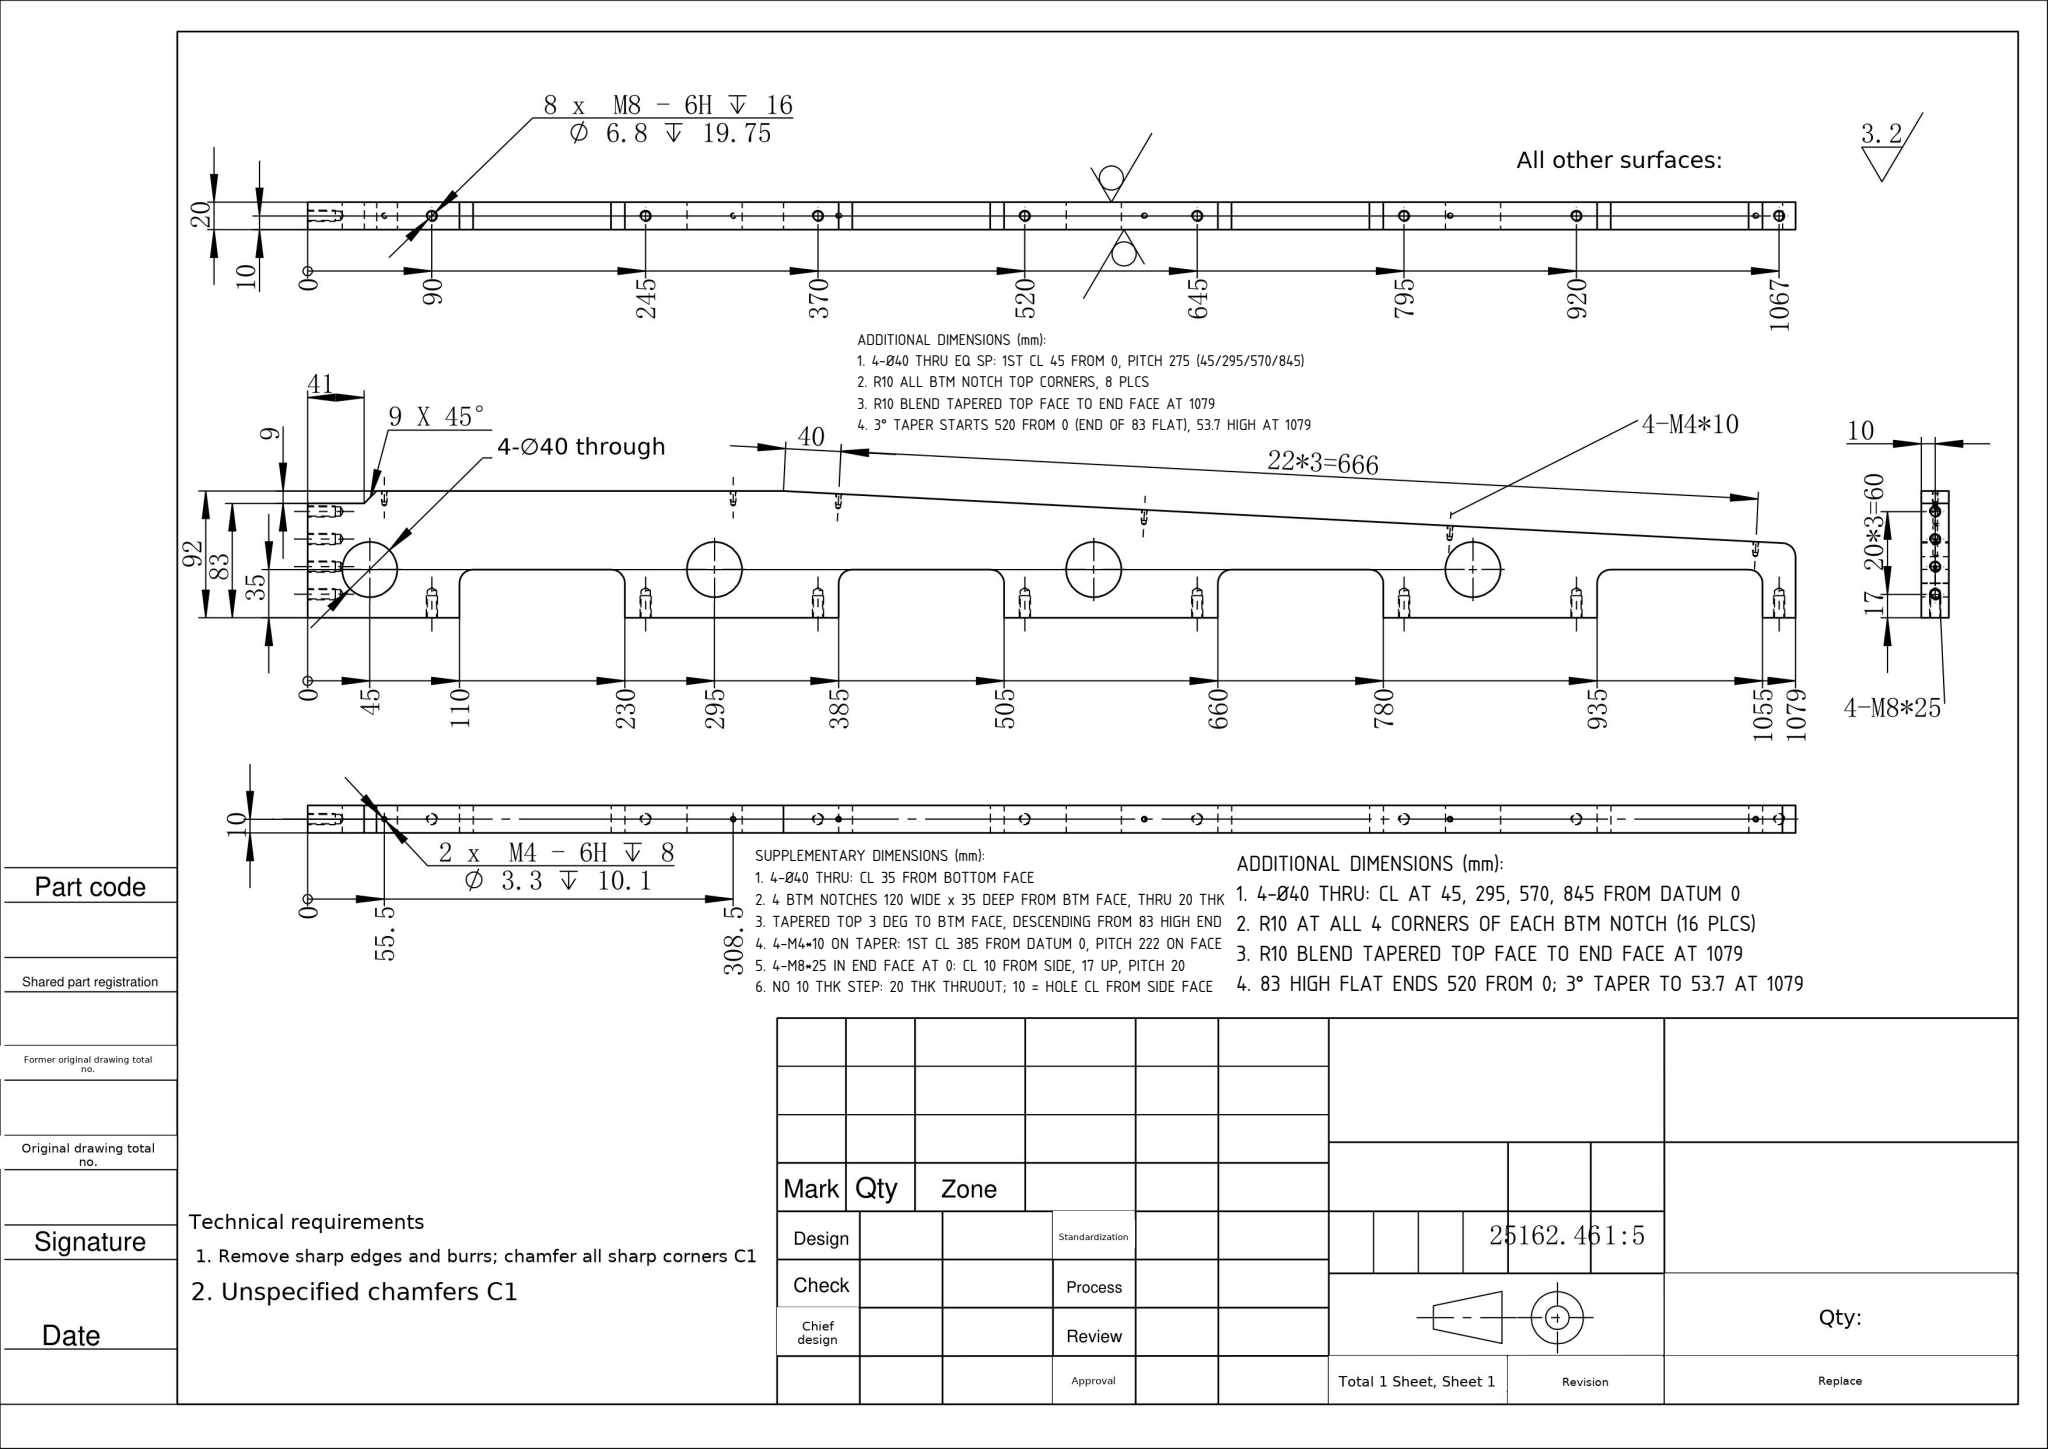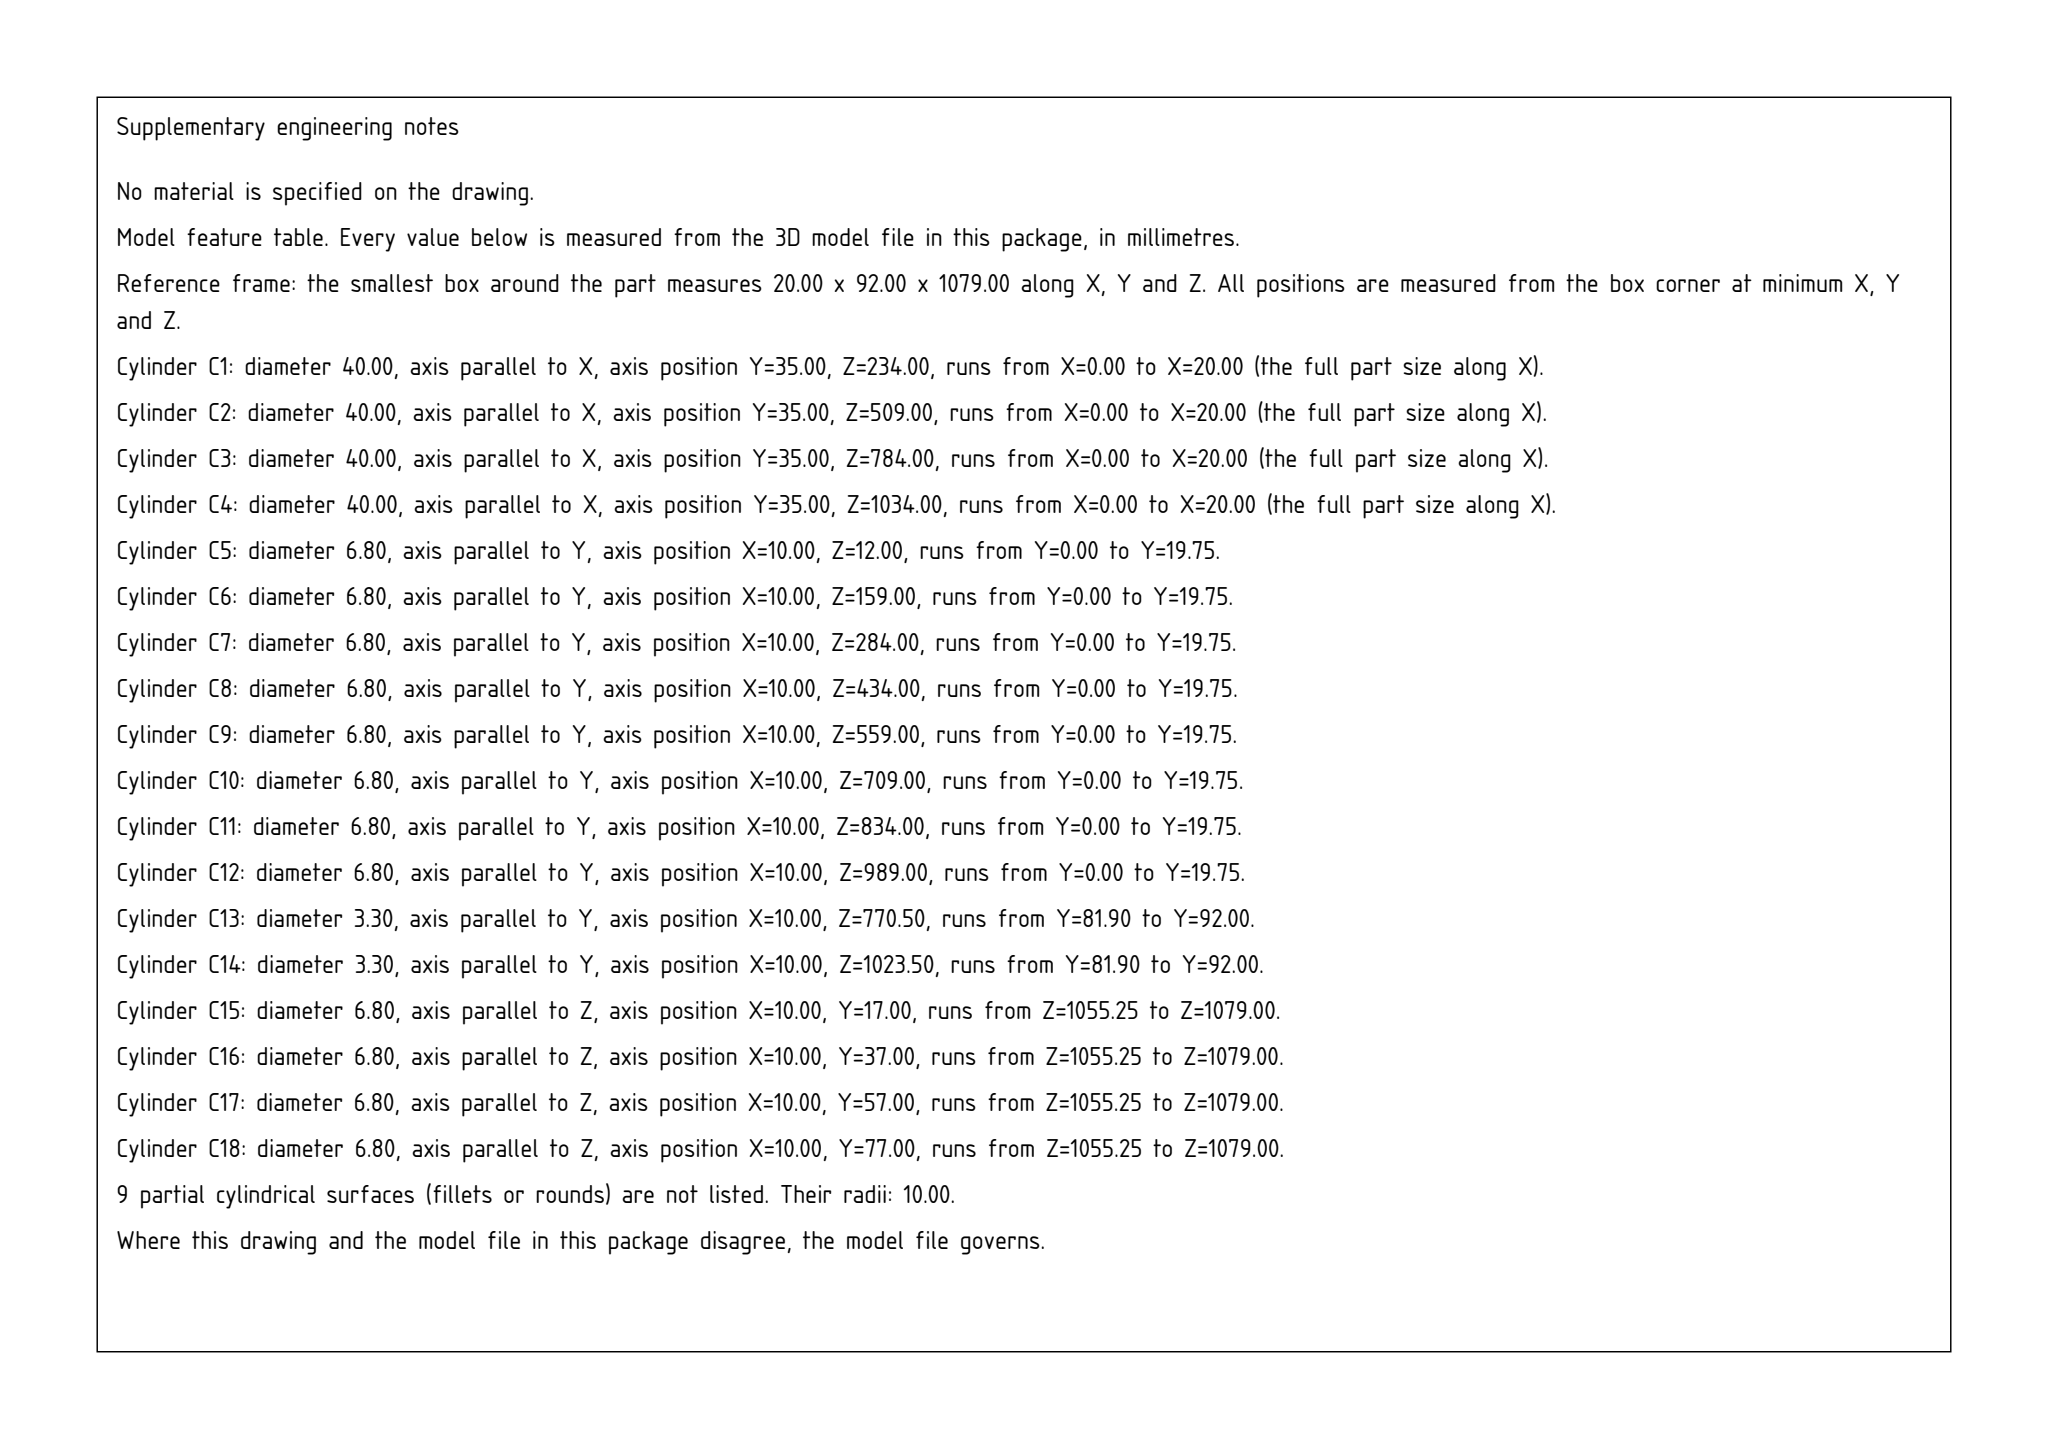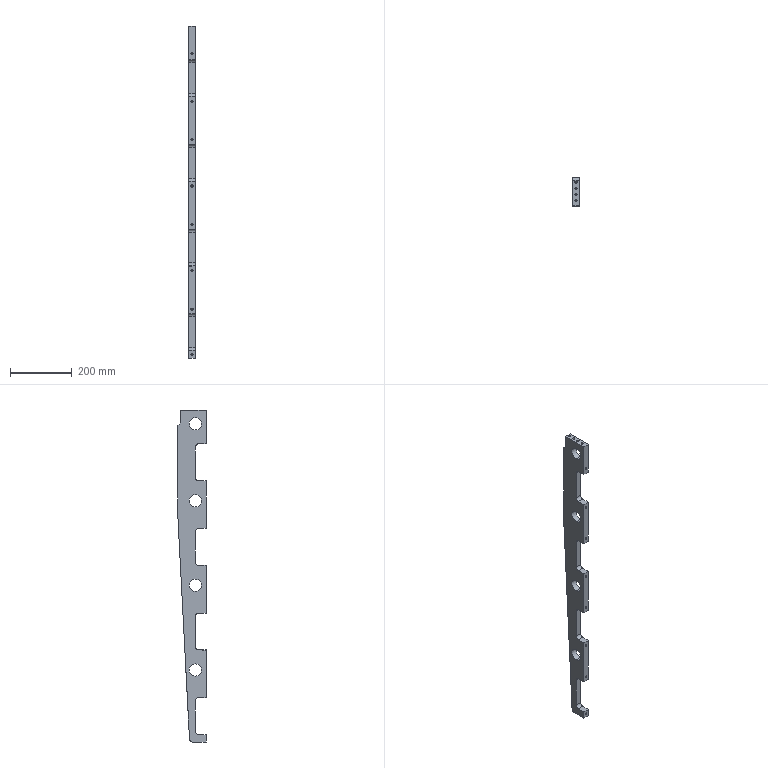Part | SolidWorks | mm | 1 solid | 114 faces | box 20 x 92 x 1079 mm | volume 1252584 mm3 | cylinder 53 | cone 36 | plane 25 | commonest cylinder face diameters 6.8 x24 3.3 x12 20 x9 40 x8